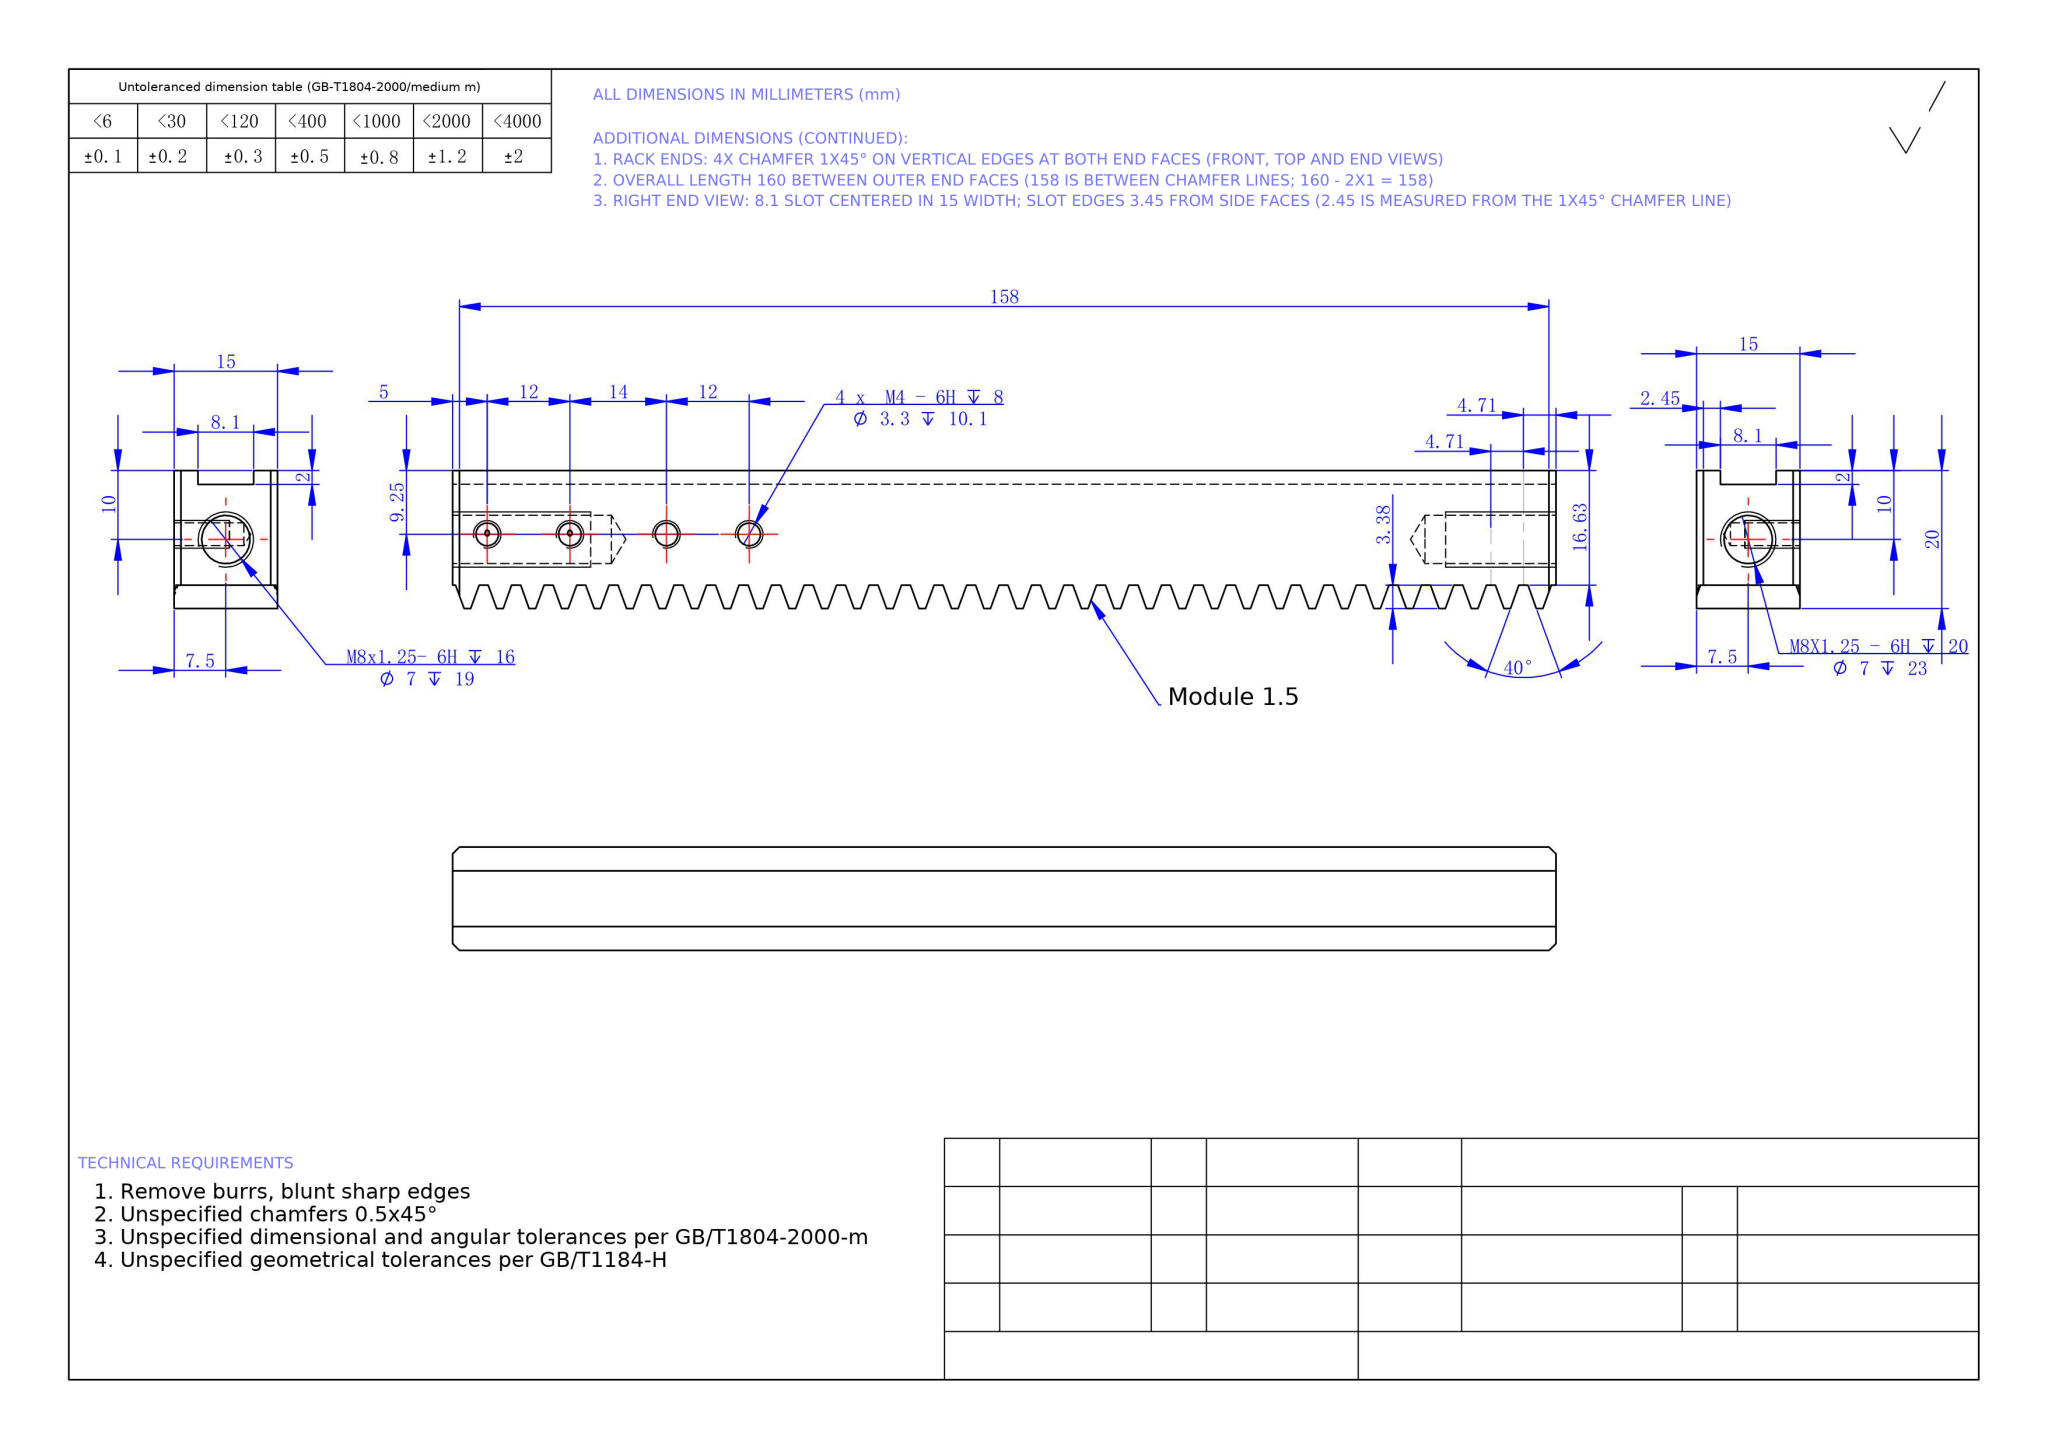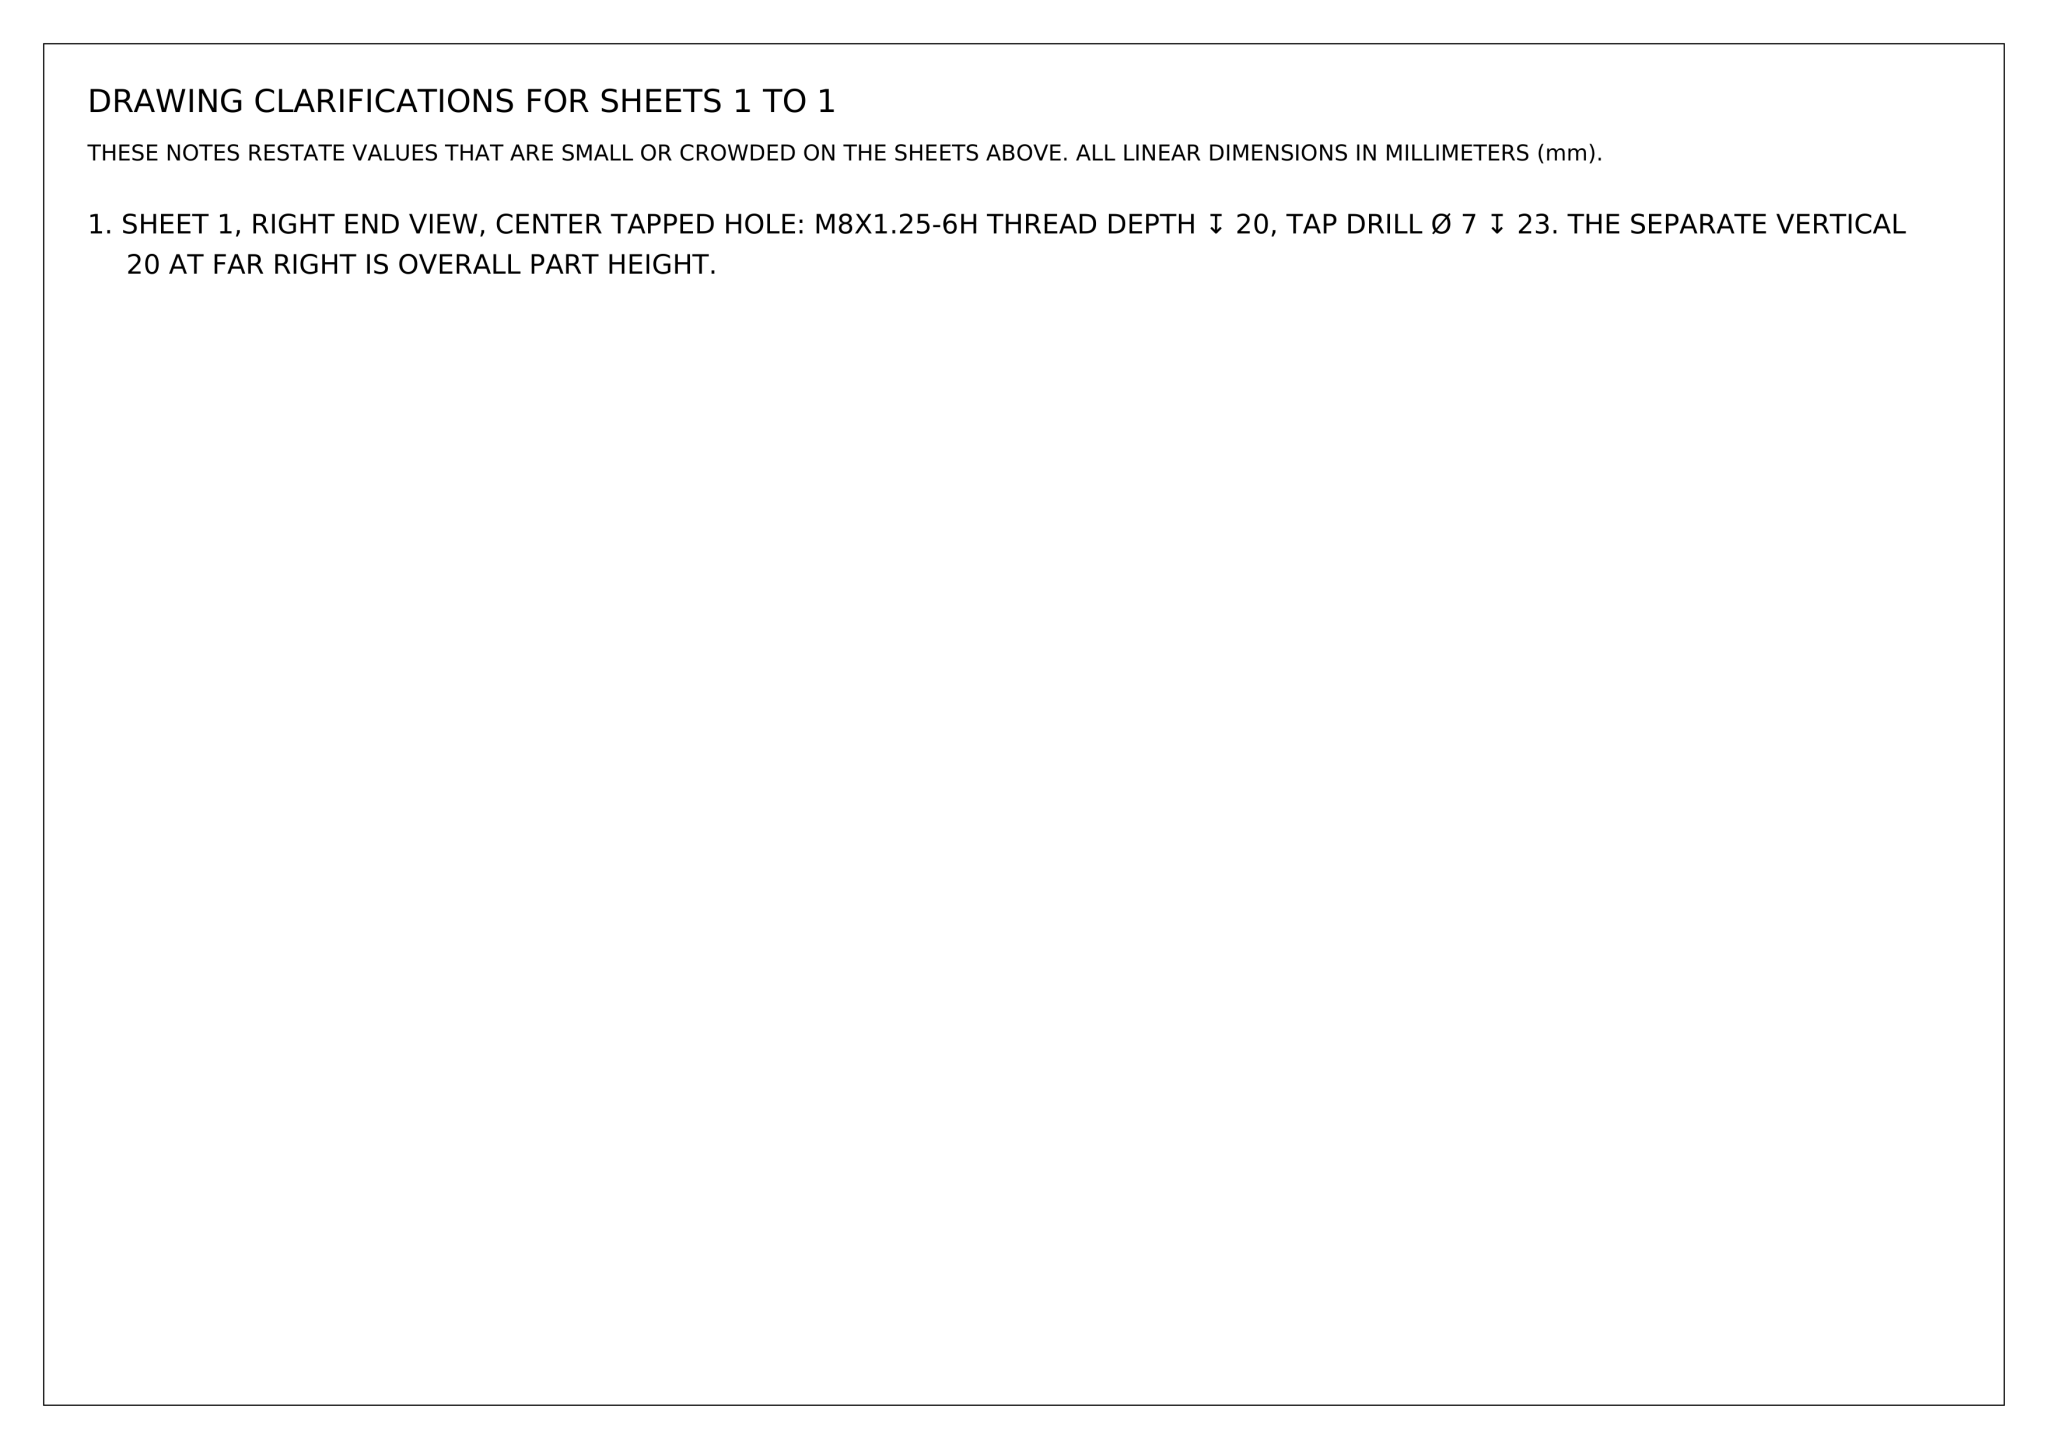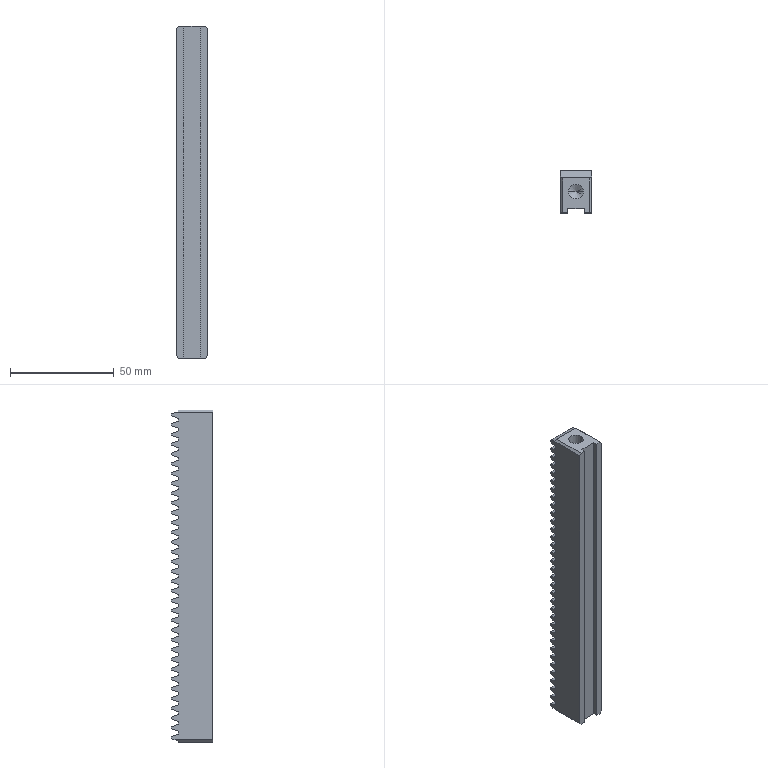Part | NX | mm | 1 solid | 178 faces | box 15 x 20 x 160 mm | volume 39097 mm3 | plane 150 | cone 14 | cylinder 14 | commonest cylinder face diameters 3.3 x10 7 x4